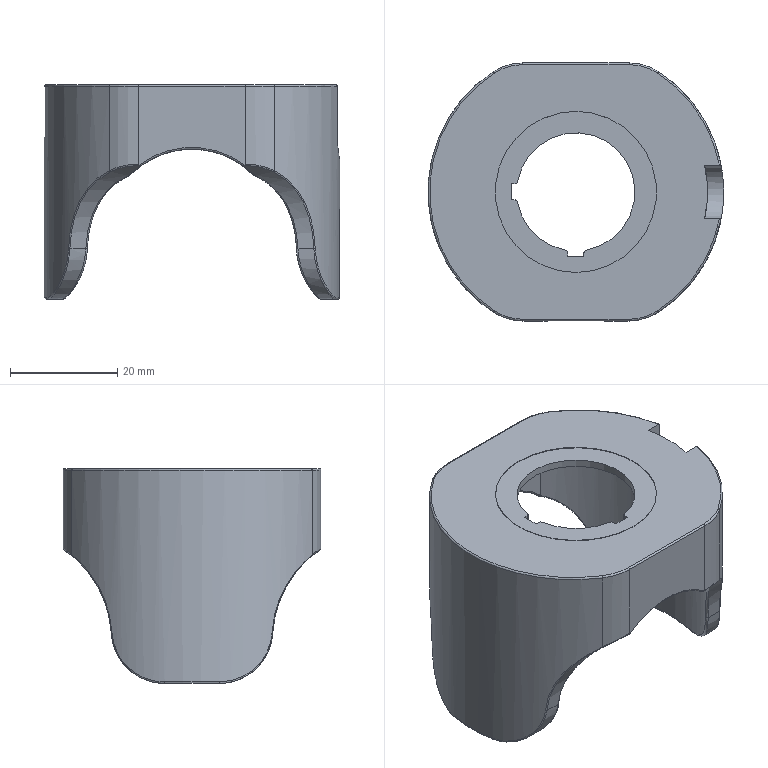Component | SolidWorks | EmergencyStopProtectiveCover-1 | 4 solids | 126 faces | volume 13879 mm3 | cylinder 50 | plane 29 | spline 24 | torus 15 | sphere 8 | commonest cylinder face diameters 0.6 x14 20 x8 47.4 x6 40 x4 1 x4 44 x3 4 x2 30 x2